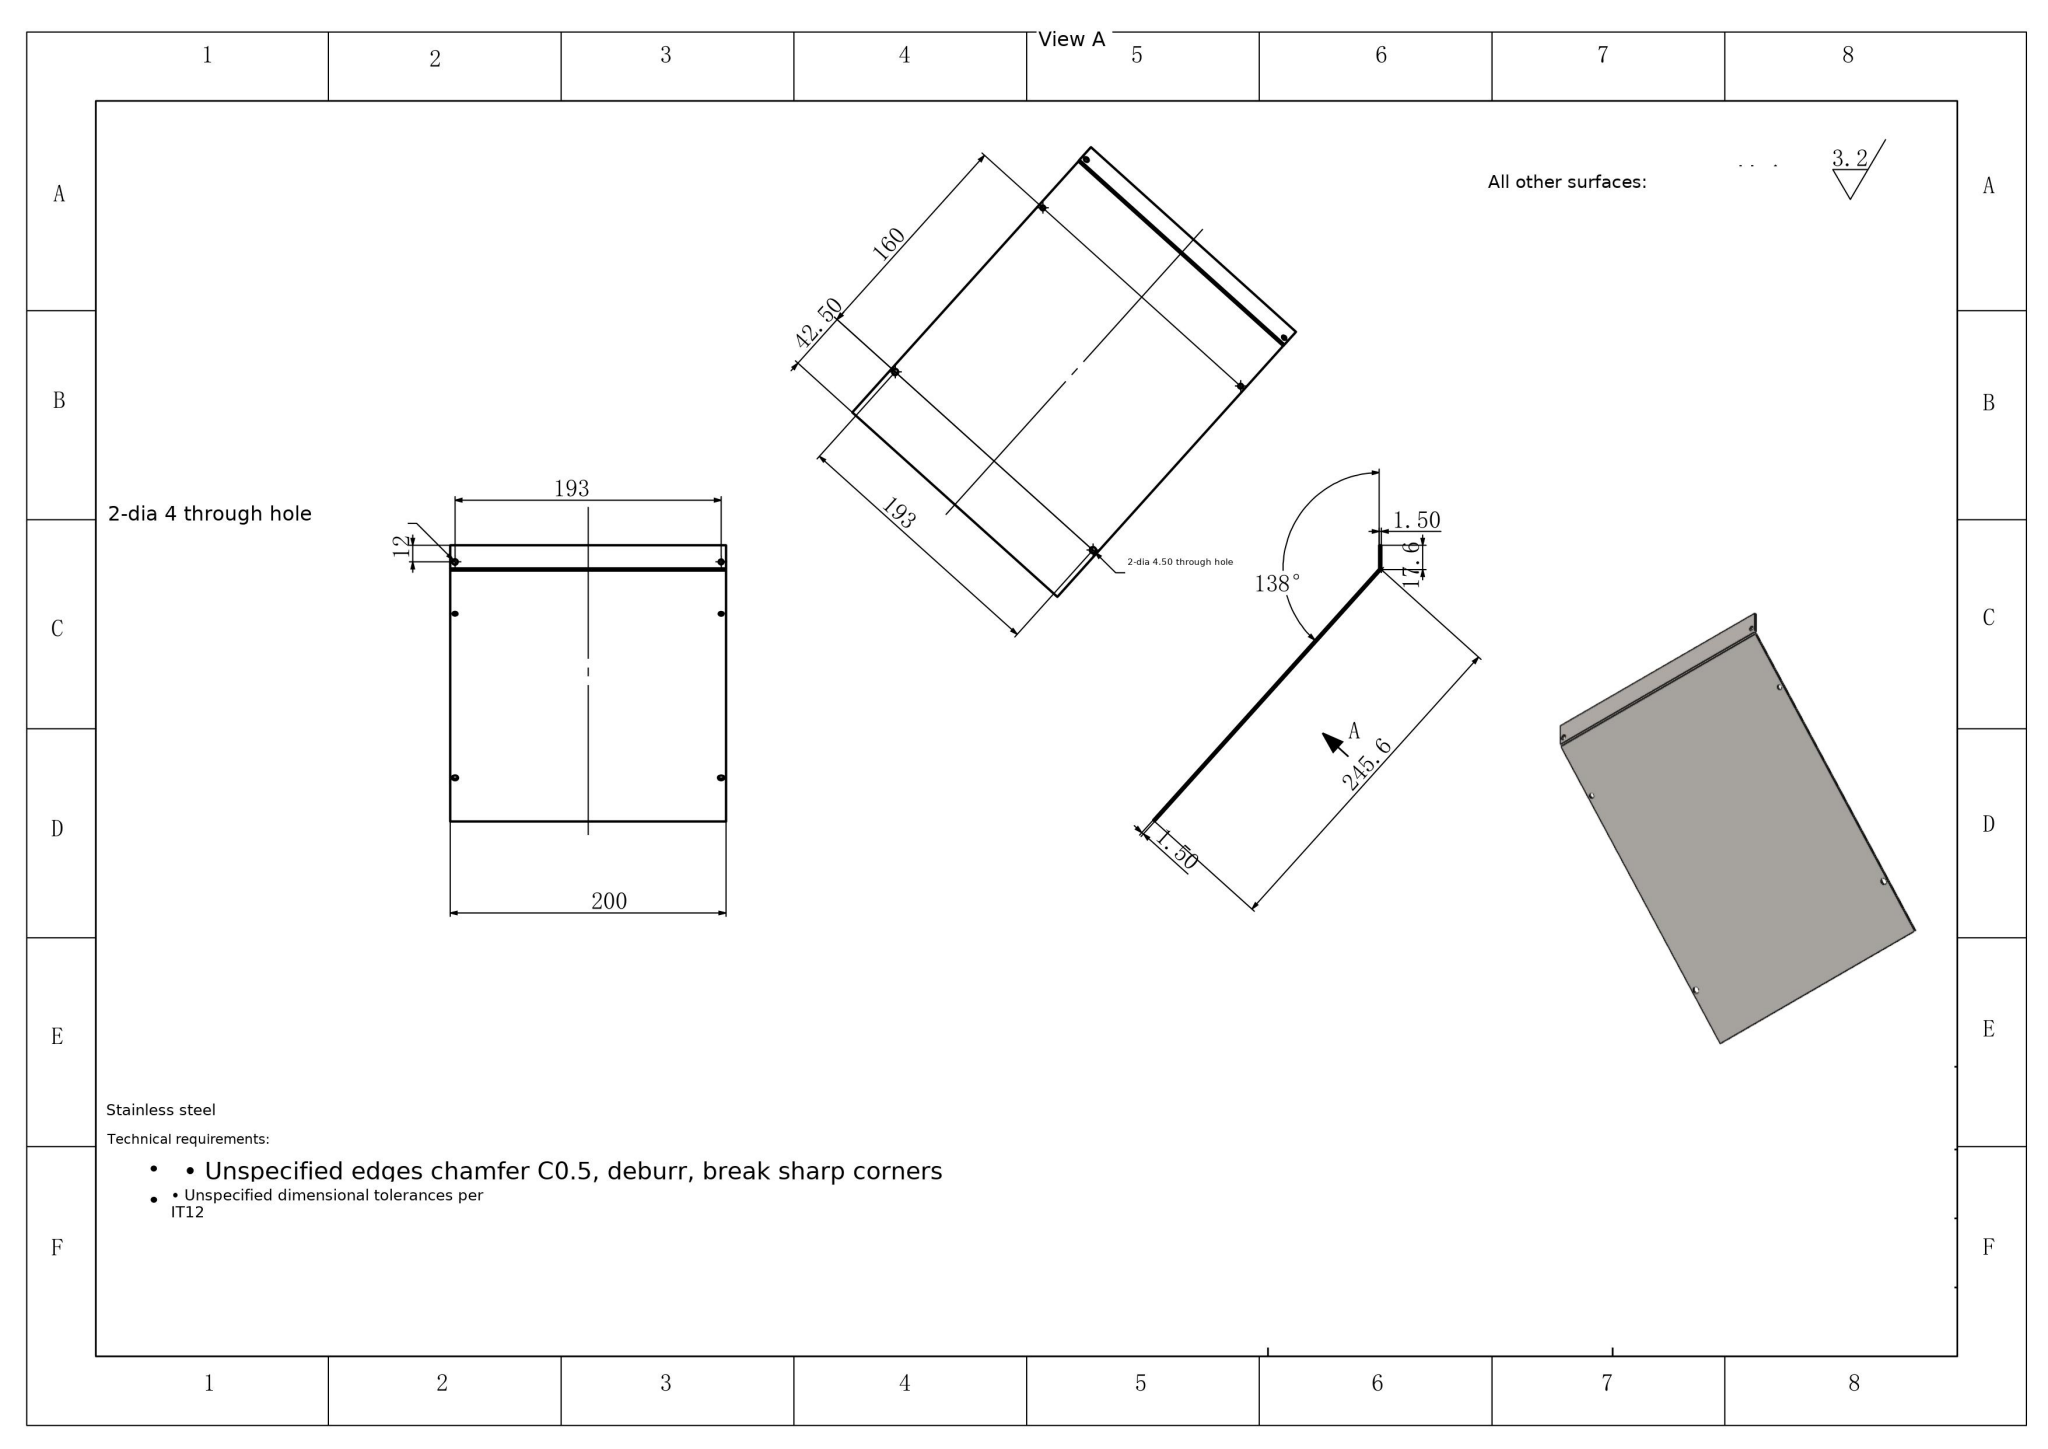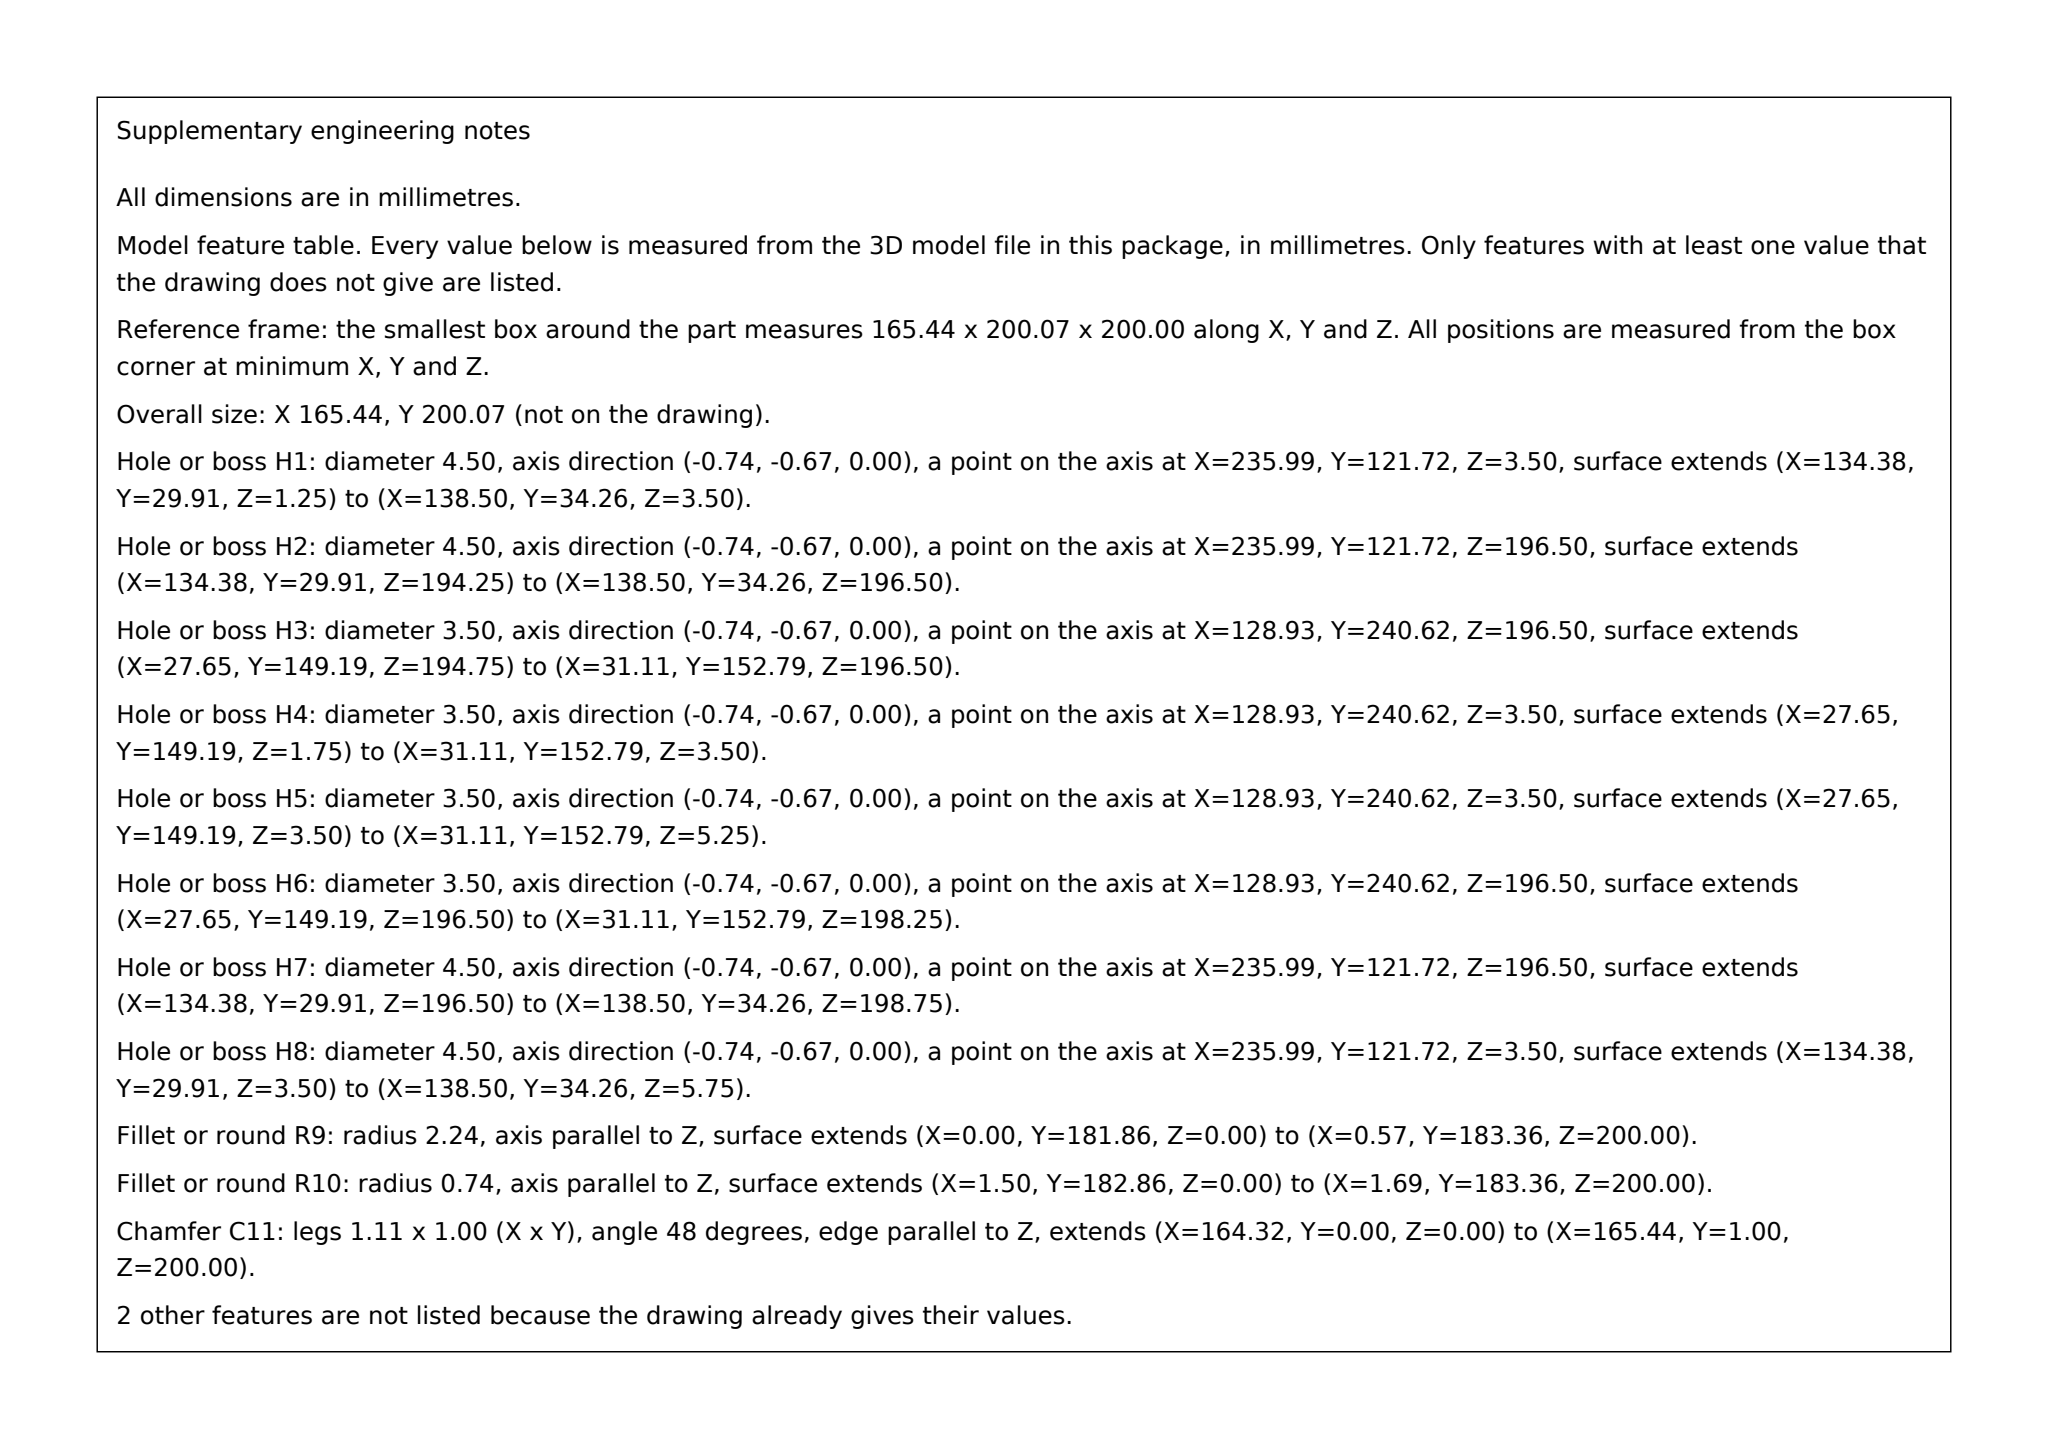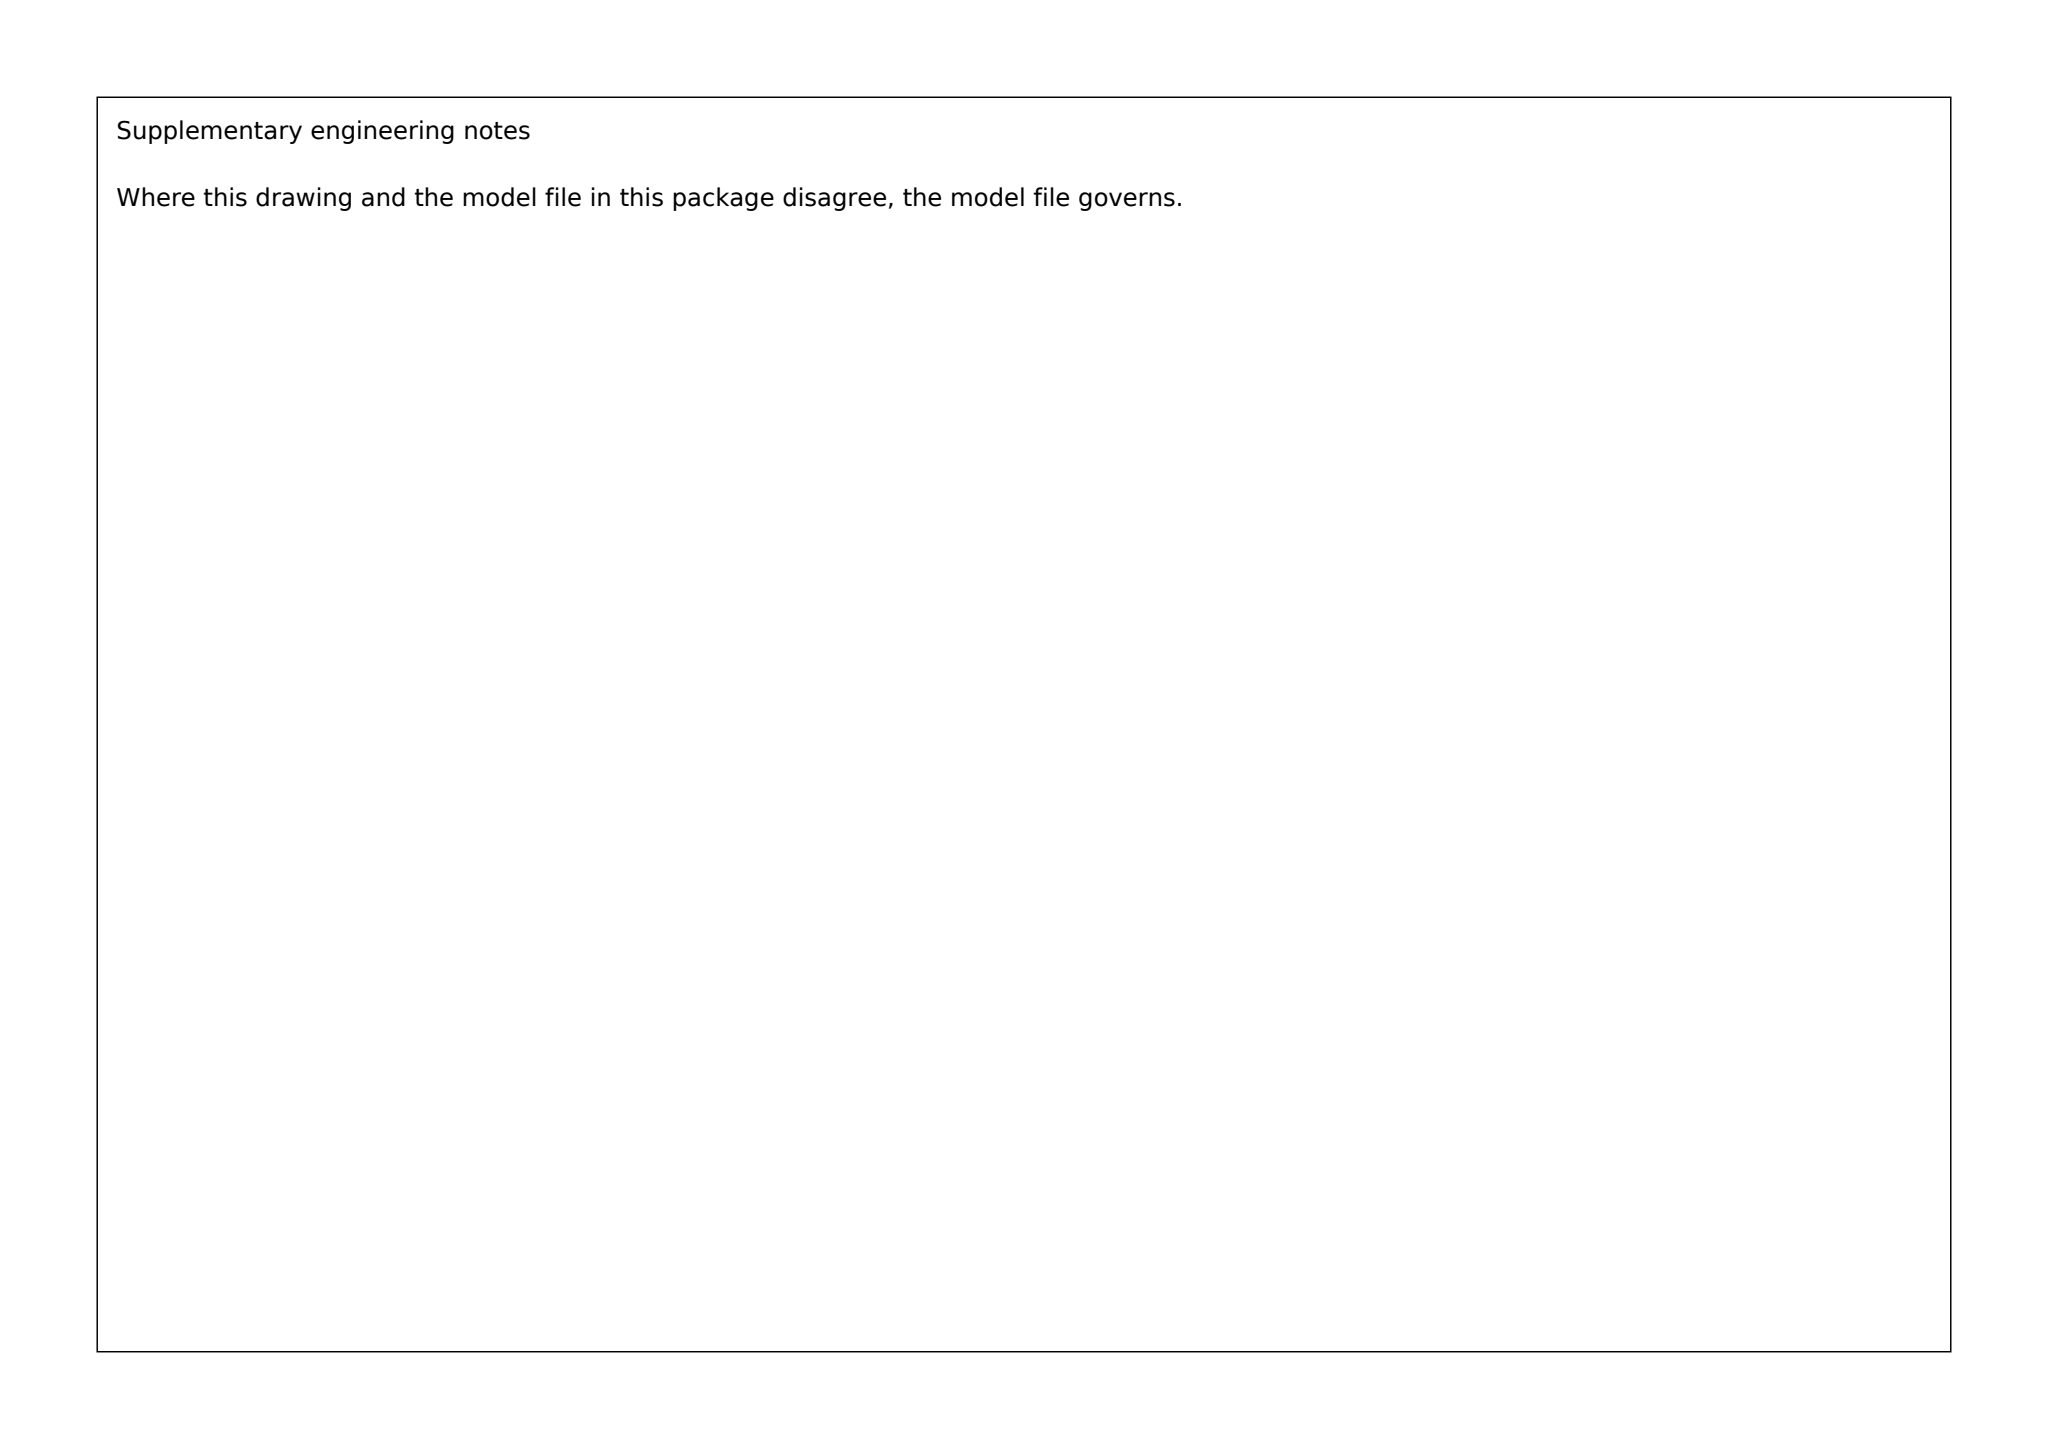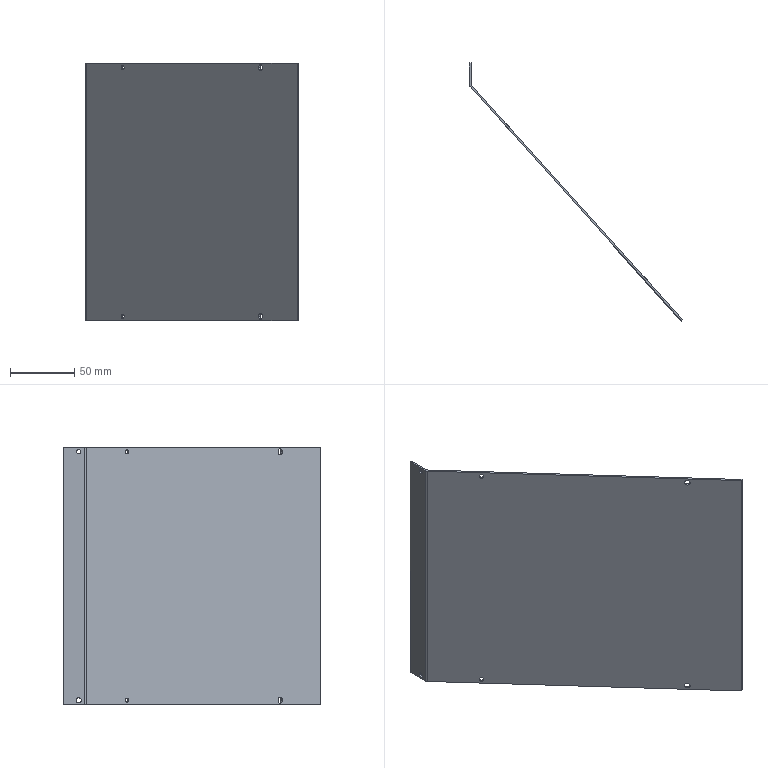Part | SolidWorks | mm | material Stainless steel | 1 solid | 26 faces | box 165.44 x 200.07 x 200 mm | volume 78647 mm3 | cylinder 14 | plane 12 | commonest cylinder face diameters 3.5 x6 4.5 x4 4 x2 1.473 x1 4.473 x1